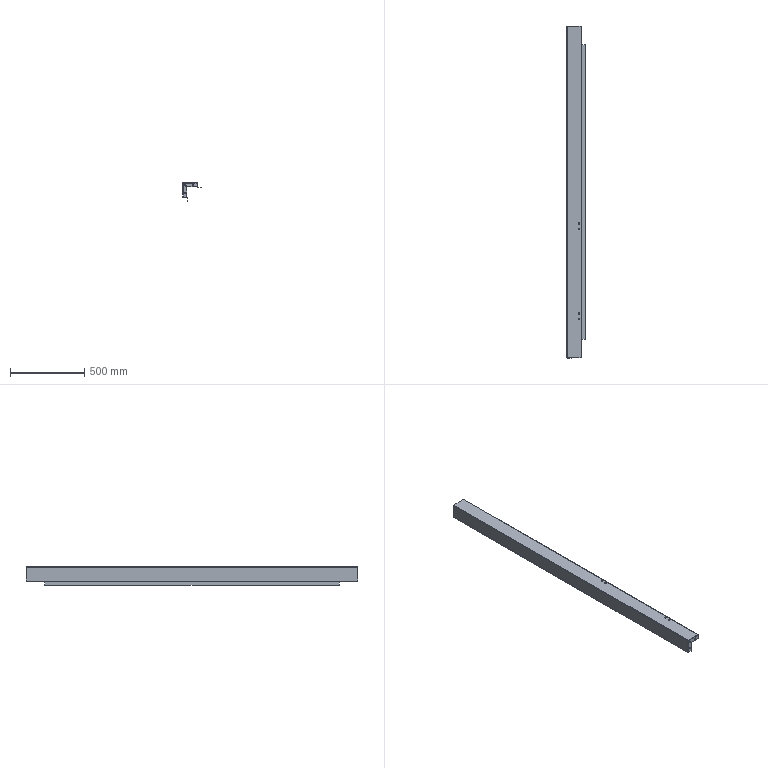Component | SolidWorks | 09LeftFrontColumn-2 | 1 solid | 133 faces | volume 1330251 mm3 | cylinder 77 | plane 54 | spline 2 | commonest cylinder face diameters 10 x59 6 x7 2 x7 9.35 x2 10.954 x2